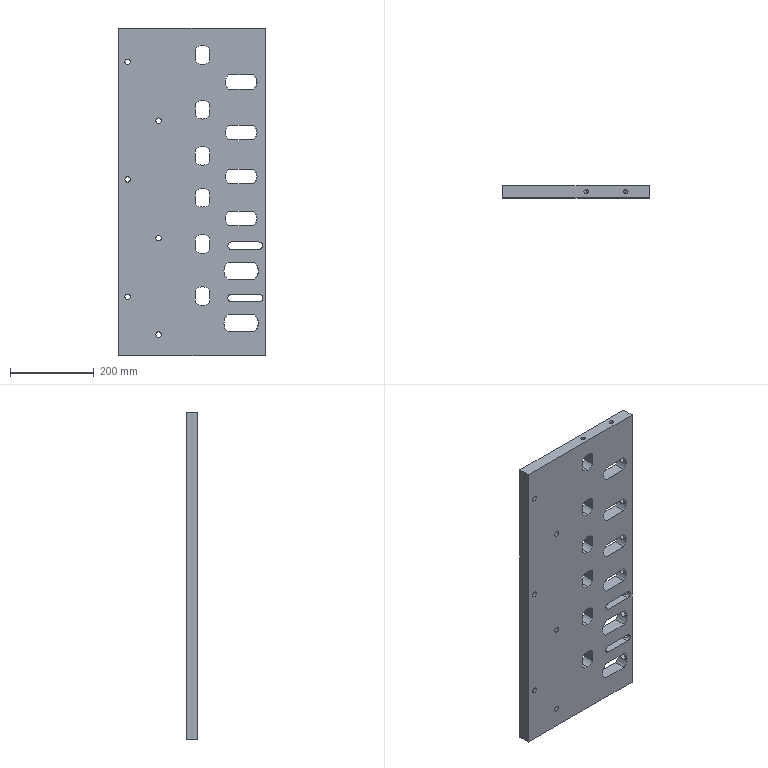Component | SolidWorks | 12ATransverseStraighteningPlatePart-2_12ATransverseStraighteningPlate-1 | 1 solid | 104 faces | box 350 x 28.5 x 780 mm | volume 6949889 mm3 | cylinder 66 | plane 34 | cone 4 | commonest cylinder face diameters 45 x26 13 x12 15.5 x8 14 x8 10.2 x4 52 x4 18 x4 | material Q235
build123d program:
from build123d import *

# Parameters (mm, degrees)
SKETCH2_W                  = 780
SKETCH2_H                  = 350
BOSS_EXTRUDE1_DEPTH        = 28.5
CUT_EXTRUDE1_DEPTH         = 429.412
CUT_EXTRUDE2_DEPTH         = 30
F_13_0_13_DIAMETER_HOLE1_D = 13
M12_TAPPED_HOLE1_D         = 10.2
M12_TAPPED_HOLE1_DEPTH     = 32.75
M12_TAPPED_HOLE1_TIP       = 3.064
M16_TAPPED_HOLE1_REACH     = 526.797
M16_TAPPED_HOLE1_BORE_R    = 7
M18_TAPPED_HOLE2_REACH     = 526.797
M18_TAPPED_HOLE2_BORE_R    = 7.75


with BuildPart() as part:
    # Sketch2 → Boss-Extrude1 (new body)
    with BuildSketch(Plane.XY):
        Rectangle(SKETCH2_W, SKETCH2_H)
    extrude(amount=BOSS_EXTRUDE1_DEPTH)

    # Sketch3 → Cut-Extrude1 (cut, through all)
    with BuildSketch(Plane.XY.offset(28.5)):
        with BuildLine():
            Line((-279.5, 146.642), (-279.5, 87.358))
            ThreePointArc((-279.5, 87.358), (-262, 79), (-244.5, 87.358))
            Line((-244.5, 87.358), (-244.5, 146.642))
            ThreePointArc((-244.5, 146.642), (-262, 155), (-279.5, 146.642))
        make_face()
        with BuildLine():
            Line((-159.5, 146.642), (-159.5, 87.358))
            ThreePointArc((-159.5, 87.358), (-142, 79), (-124.5, 87.358))
            Line((-124.5, 87.358), (-124.5, 146.642))
            ThreePointArc((-124.5, 146.642), (-142, 155), (-159.5, 146.642))
        make_face()
        with BuildLine():
            Line((-19.5, 146.642), (-19.5, 87.358))
            ThreePointArc((-19.5, 87.358), (-37, 79), (-54.5, 87.358))
            Line((-54.5, 87.358), (-54.5, 146.642))
            ThreePointArc((-54.5, 146.642), (-37, 155), (-19.5, 146.642))
        make_face()
        with BuildLine():
            Line((80.5, 146.642), (80.5, 87.358))
            ThreePointArc((80.5, 87.358), (63, 79), (45.5, 87.358))
            Line((45.5, 87.358), (45.5, 146.642))
            ThreePointArc((45.5, 146.642), (63, 155), (80.5, 146.642))
        make_face()
        with BuildLine():
            Line((167.5, 147.992), (167.5, 86.008))
            ThreePointArc((167.5, 86.008), (188, 76), (208.5, 86.008))
            Line((208.5, 86.008), (208.5, 147.992))
            ThreePointArc((208.5, 147.992), (188, 158), (167.5, 147.992))
        make_face()
        with BuildLine():
            Line((333.5, 147.992), (333.5, 86.008))
            ThreePointArc((333.5, 86.008), (313, 76), (292.5, 86.008))
            Line((292.5, 86.008), (292.5, 147.992))
            ThreePointArc((292.5, 147.992), (313, 158), (333.5, 147.992))
        make_face()
        with BuildLine():
            Line((137, 159.5), (137, 94.5))
            ThreePointArc((137, 94.5), (128, 85.5), (119, 94.5))
            Line((119, 94.5), (119, 159.5))
            ThreePointArc((119, 159.5), (128, 168.5), (137, 159.5))
        make_face()
        with BuildLine():
            Line((262, 159.5), (262, 94.5))
            ThreePointArc((262, 94.5), (253, 85.5), (244, 94.5))
            Line((244, 94.5), (244, 159.5))
            ThreePointArc((244, 159.5), (253, 168.5), (262, 159.5))
        make_face()
    extrude(amount=-CUT_EXTRUDE1_DEPTH, mode=Mode.SUBTRACT)

    # Sketch4 → Cut-Extrude2 (cut)
    with BuildSketch(Plane.XY.offset(28.5)):
        with BuildLine():
            Line((-340.642, 42.5), (-312.358, 42.5))
            ThreePointArc((-312.358, 42.5), (-304, 25), (-312.358, 7.5))
            Line((-312.358, 7.5), (-340.642, 7.5))
            ThreePointArc((-340.642, 7.5), (-349, 25), (-340.642, 42.5))
        make_face()
        with BuildLine():
            Line((-210.642, 7.5), (-182.358, 7.5))
            ThreePointArc((-182.358, 7.5), (-174, 25), (-182.358, 42.5))
            Line((-182.358, 42.5), (-210.642, 42.5))
            ThreePointArc((-210.642, 42.5), (-219, 25), (-210.642, 7.5))
        make_face()
        with BuildLine():
            Line((-100.642, 42.5), (-72.358, 42.5))
            ThreePointArc((-72.358, 42.5), (-64, 25), (-72.358, 7.5))
            Line((-72.358, 7.5), (-100.642, 7.5))
            ThreePointArc((-100.642, 7.5), (-109, 25), (-100.642, 42.5))
        make_face()
        with BuildLine():
            Line((-0.6421, 7.5), (27.642, 7.5))
            ThreePointArc((27.642, 7.5), (36, 25), (27.642, 42.5))
            Line((27.642, 42.5), (-0.6421, 42.5))
            ThreePointArc((-0.6421, 42.5), (-9, 25), (-0.6421, 7.5))
        make_face()
        with BuildLine():
            Line((109.358, 42.5), (137.642, 42.5))
            ThreePointArc((137.642, 42.5), (146, 25), (137.642, 7.5))
            Line((137.642, 7.5), (109.358, 7.5))
            ThreePointArc((109.358, 7.5), (101, 25), (109.358, 42.5))
        make_face()
        with BuildLine():
            Line((234.358, 42.5), (262.642, 42.5))
            ThreePointArc((262.642, 42.5), (271, 25), (262.642, 7.5))
            Line((262.642, 7.5), (234.358, 7.5))
            ThreePointArc((234.358, 7.5), (226, 25), (234.358, 42.5))
        make_face()
    extrude(amount=-CUT_EXTRUDE2_DEPTH, mode=Mode.SUBTRACT)

    # 13.0 _13_ Diameter Hole1 (through all)
    with Locations(Plane.XY.offset(28.5)):
        with Locations((-170, -79.5), (110, -79.5), (340, -79.5), (-310, -153.5), (-30, -153.5), (250, -153.5)):
            Hole(F_13_0_13_DIAMETER_HOLE1_D / 2)

    # M12 Tapped Hole1
    with Locations(Plane.ZY.offset(390)):
        with Locations((14.25, 24), (14.25, 119)):
            Hole(M12_TAPPED_HOLE1_D / 2, depth=M12_TAPPED_HOLE1_DEPTH)
            with Locations((0, 0, -(M12_TAPPED_HOLE1_DEPTH + M12_TAPPED_HOLE1_TIP / 2))):  # 118° drill point
                Cone(0, M12_TAPPED_HOLE1_D / 2, M12_TAPPED_HOLE1_TIP, mode=Mode.SUBTRACT)

    # M16 Tapped Hole1 bore → M16 Tapped Hole1 (cut, up to next)
    with BuildSketch(Plane(origin=(0, 175, 0), x_dir=(1, 0, 0), z_dir=(0, 1, 0)), mode=Mode.PRIVATE) as m16_tapped_hole1_sk1:
        with Locations((-262, -14.25)):
            Circle(M16_TAPPED_HOLE1_BORE_R)
    m16_tapped_hole1_tool1 = extrude(m16_tapped_hole1_sk1.sketch, amount=-M16_TAPPED_HOLE1_REACH, mode=Mode.PRIVATE) & part.part
    # M16 Tapped Hole1 bore → M16 Tapped Hole1 (cut, up to next)
    with BuildSketch(Plane(origin=(0, 175, 0), x_dir=(1, 0, 0), z_dir=(0, 1, 0)), mode=Mode.PRIVATE) as m16_tapped_hole1_sk2:
        with Locations((-142, -14.25)):
            Circle(M16_TAPPED_HOLE1_BORE_R)
    m16_tapped_hole1_tool2 = extrude(m16_tapped_hole1_sk2.sketch, amount=-M16_TAPPED_HOLE1_REACH, mode=Mode.PRIVATE) & part.part
    # M16 Tapped Hole1 bore → M16 Tapped Hole1 (cut, up to next)
    with BuildSketch(Plane(origin=(0, 175, 0), x_dir=(1, 0, 0), z_dir=(0, 1, 0)), mode=Mode.PRIVATE) as m16_tapped_hole1_sk3:
        with Locations((-37, -14.25)):
            Circle(M16_TAPPED_HOLE1_BORE_R)
    m16_tapped_hole1_tool3 = extrude(m16_tapped_hole1_sk3.sketch, amount=-M16_TAPPED_HOLE1_REACH, mode=Mode.PRIVATE) & part.part
    # M16 Tapped Hole1 bore → M16 Tapped Hole1 (cut, up to next)
    with BuildSketch(Plane(origin=(0, 175, 0), x_dir=(1, 0, 0), z_dir=(0, 1, 0)), mode=Mode.PRIVATE) as m16_tapped_hole1_sk4:
        with Locations((63, -14.25)):
            Circle(M16_TAPPED_HOLE1_BORE_R)
    m16_tapped_hole1_tool4 = extrude(m16_tapped_hole1_sk4.sketch, amount=-M16_TAPPED_HOLE1_REACH, mode=Mode.PRIVATE) & part.part
    add(m16_tapped_hole1_tool1.solids().sort_by_distance((-262, 175, 14.25))[0], mode=Mode.SUBTRACT)
    add(m16_tapped_hole1_tool2.solids().sort_by_distance((-142, 175, 14.25))[0], mode=Mode.SUBTRACT)
    add(m16_tapped_hole1_tool3.solids().sort_by_distance((-37, 175, 14.25))[0], mode=Mode.SUBTRACT)
    add(m16_tapped_hole1_tool4.solids().sort_by_distance((63, 175, 14.25))[0], mode=Mode.SUBTRACT)

    # M18 Tapped Hole2 bore → M18 Tapped Hole2 (cut, up to next)
    with BuildSketch(Plane(origin=(0, 175, 0), x_dir=(1, 0, 0), z_dir=(0, 1, 0)), mode=Mode.PRIVATE) as m18_tapped_hole2_sk1:
        with Locations((253, -14.25)):
            Circle(M18_TAPPED_HOLE2_BORE_R)
    m18_tapped_hole2_tool1 = extrude(m18_tapped_hole2_sk1.sketch, amount=-M18_TAPPED_HOLE2_REACH, mode=Mode.PRIVATE) & part.part
    # M18 Tapped Hole2 bore → M18 Tapped Hole2 (cut, up to next)
    with BuildSketch(Plane(origin=(0, 175, 0), x_dir=(1, 0, 0), z_dir=(0, 1, 0)), mode=Mode.PRIVATE) as m18_tapped_hole2_sk2:
        with Locations((188, -14.25)):
            Circle(M18_TAPPED_HOLE2_BORE_R)
    m18_tapped_hole2_tool2 = extrude(m18_tapped_hole2_sk2.sketch, amount=-M18_TAPPED_HOLE2_REACH, mode=Mode.PRIVATE) & part.part
    # M18 Tapped Hole2 bore → M18 Tapped Hole2 (cut, up to next)
    with BuildSketch(Plane(origin=(0, 175, 0), x_dir=(1, 0, 0), z_dir=(0, 1, 0)), mode=Mode.PRIVATE) as m18_tapped_hole2_sk3:
        with Locations((128, -14.25)):
            Circle(M18_TAPPED_HOLE2_BORE_R)
    m18_tapped_hole2_tool3 = extrude(m18_tapped_hole2_sk3.sketch, amount=-M18_TAPPED_HOLE2_REACH, mode=Mode.PRIVATE) & part.part
    # M18 Tapped Hole2 bore → M18 Tapped Hole2 (cut, up to next)
    with BuildSketch(Plane(origin=(0, 175, 0), x_dir=(1, 0, 0), z_dir=(0, 1, 0)), mode=Mode.PRIVATE) as m18_tapped_hole2_sk4:
        with Locations((313, -14.25)):
            Circle(M18_TAPPED_HOLE2_BORE_R)
    m18_tapped_hole2_tool4 = extrude(m18_tapped_hole2_sk4.sketch, amount=-M18_TAPPED_HOLE2_REACH, mode=Mode.PRIVATE) & part.part
    add(m18_tapped_hole2_tool1.solids().sort_by_distance((253, 175, 14.25))[0], mode=Mode.SUBTRACT)
    add(m18_tapped_hole2_tool2.solids().sort_by_distance((188, 175, 14.25))[0], mode=Mode.SUBTRACT)
    add(m18_tapped_hole2_tool3.solids().sort_by_distance((128, 175, 14.25))[0], mode=Mode.SUBTRACT)
    add(m18_tapped_hole2_tool4.solids().sort_by_distance((313, 175, 14.25))[0], mode=Mode.SUBTRACT)


solid = part.part

# Placed as in the assembly
solid = solid.moved(Location((87.617, 155.96, 176), (90, 0, -90)))